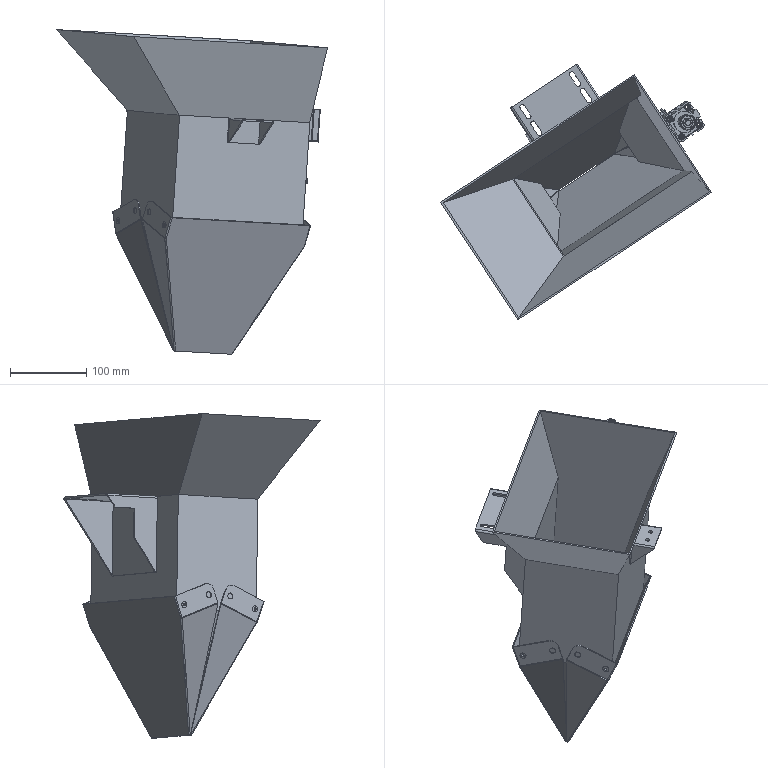Assembly | SolidWorks | mm | 21 component files | 21 solids | 784 faces | box 355.68 x 336.06 x 426.21 mm | volume 669723 mm3 | plane 339 | cylinder 308 | cone 109 | spline 16 | torus 10 | sphere 2 | commonest cylinder face diameters 8 x60 0.4 x46 7.9 x18 8.2 x16 4.917 x16 0.2 x12 6.5 x12 3.2 x9
Bill of materials:
BucketCylinderConnection | 1 | AISI 304 | Thin-wall formed bracket: a rectangular plate with four elongated slots, and side walls bent down along two opposite edges. The side walls have tapered, non-rectangular outlines.
DoorConnectionPiece | 2 | AISI 304 | Flat elongated link or strap with fully rounded ends and one round through-hole near each end.
DoorCylinderMount | 1 | AISI 304 | Thin L-shaped angle bracket. One leg is plain and rectangular. The other leg has a large central hole with four smaller holes arranged around it.
DoorFisheyeShaftPin | 1 |  | Headed bolt-like pin: a short head with flat faces on its sides, a plain cylindrical shank, and a section of external thread-like grooves at the free end.
DoorGasket | 4 |  | Plain cylindrical sleeve or spacer with a concentric round through-bore and flat ends.
F-M8X125U | 1 |  | Rod-end-style eye component: a rounded eye housing holding a separate-looking ring with a bore, a cylindrical shank, and a hexagonal collar with an axial bore at the end of the shank.
KnucklePin | 2 |  | Flanged bushing: a cylindrical body with a concentric through-bore, and a larger flange at one end that has at least one straight flat on its edge.
LinearGuideRodSheetMetal | 1 | AISI 304 | Thin formed channel-type bracket: a rectangular base plate with two round holes, and triangular walls bent up along two opposite edges.
MaterialChannel | 1 | AISI 304 | Thin open sheet-metal shape like a hopper or chute: an outward-flared rectangular upper rim, vertical walls below it, and tapered tabs or legs hanging from the lower edge.
MaterialGate | 2 | AISI 304 | Tapered open trough: a trapezoidal bottom panel with two inclined side walls narrowing toward one end. At the wide end there are bent-out end tabs, each with two round holes.
SDAJ-25x20_20b | 1 |  | Compact, roughly square prismatic block with chamfered corners and lengthwise extruded-profile grooves on its sides. Each end face has four corner through-holes with counterbores, a shallow circular recess or ring, and a raised central cylindrical boss with a central bore. The boss sticks out a little from both end faces. One side face has two small round ports.
Mates:
1. coincident | MaterialGate-1 face at (-298.666, 15.944, 688.726) dir (-0.8341, -0.5496, 0.04788) | MaterialGate-2 face at (-295.771, 11.528, 688.461) dir (-0.8341, -0.5496, 0.04788)
2. coincident | DoorConnectionPiece-1 face at (-101.704, 138.808, 740.065) dir (-0.8341, -0.5496, 0.04788) | DoorConnectionPiece-2 face at (-101.704, 138.808, 740.065) dir (0.8341, 0.5496, -0.04788)
3. concentric | KnucklePin-2 face at (-94.22, 126.738, 686.887) dir (-0.8341, -0.5496, 0.04788) r 4 | DoorConnectionPiece-1 face at (-96.017, 125.554, 686.99) dir (0.8341, 0.5496, -0.04788) r 4
4. concentric | KnucklePin-1 face at (-112.662, 154.873, 688.573) dir (-0.8341, -0.5496, 0.04788) r 4 | DoorConnectionPiece-2 face at (-116.128, 152.59, 688.772) dir (0.8341, 0.5496, -0.04788) r 4
5. coincident | MaterialChannel-1 face at (-315.723, 67.887, 831.179) dir (-0.5475, 0.8353, 0.05005) | BucketCylinderConnection-1 face at (-274.02, 95.366, 828.785) dir (0.5475, -0.8353, -0.05005)
6. coincident | MaterialChannel-1 face at (-144.74, 180.552, 821.364) dir (0.8341, 0.5496, -0.04788) | DoorCylinderMount-1 face at (-123.09, 145.425, 795.294) dir (-0.8341, -0.5496, 0.04788)
7. distance | BucketCylinderConnection-1 face at (-229.15, 218.226, 827.661) dir (0.8341, 0.5496, -0.04788) | MaterialChannel-1 face at (-144.74, 180.552, 821.364) dir (0.8341, 0.5496, -0.04788)
8. distance | DoorCylinderMount-1 face at (-99.938, 112.837, 793.221) dir (0.5475, -0.8353, -0.05005) | MaterialChannel-1 face at (-247.283, -36.525, 824.923) dir (0.5475, -0.8353, -0.05005)
9. coincident | MaterialChannel-1 face at (-315.723, 67.887, 831.179) dir (0.0675, -0.01553, 0.9976) | BucketCylinderConnection-1 face at (-229.15, 218.226, 827.661) dir (0.0675, -0.01553, 0.9976)
10. concentric | MaterialChannel-1 face at (-89.92, 84.239, 670.806) dir (-0.8341, -0.5496, 0.04788) r 4 | MaterialGate-2 face at (-84.915, 87.537, 670.519) dir (0.8341, 0.5496, -0.04788) r 4
11. concentric | MaterialChannel-1 face at (-150.695, 176.957, 676.362) dir (-0.8341, -0.5496, 0.04788) r 4 | MaterialGate-1 face at (-145.69, 180.254, 676.074) dir (0.8341, 0.5496, -0.04788) r 4
12. coincident | MaterialChannel-1 face at (-247.283, -36.525, 824.923) dir (0.5475, -0.8353, -0.05005) | LinearGuideRodSheetMetal-1 face at (-182.778, 6.099, 819.217) dir (-0.5475, 0.8353, 0.05005)
13. coincident | BucketCylinderConnection-1 face at (-229.15, 218.226, 827.661) dir (0.0675, -0.01553, 0.9976) | LinearGuideRodSheetMetal-1 face at (-181.548, 4.398, 821.112) dir (0.0675, -0.01553, 0.9976)
14. distance | MaterialChannel-1 face at (-144.74, 180.552, 821.364) dir (0.8341, 0.5496, -0.04788) | MaterialGate-1 face at (-116.423, 136.028, 678.264) dir (-0.8341, -0.5496, 0.04788)
15. distance | LinearGuideRodSheetMetal-1 face at (-181.683, 4.429, 819.117) dir (-0.8341, -0.5496, 0.04788) | MaterialChannel-1 face at (-315.723, 67.887, 831.179) dir (-0.8341, -0.5496, 0.04788)
16. concentric | MaterialChannel-1 face at (-89.92, 84.239, 670.806) dir (-0.8341, -0.5496, 0.04788) r 4 | DoorGasket-1 face at (-259.235, -27.327, 680.526) dir (-0.8341, -0.5496, 0.04788) r 4
17. concentric | MaterialChannel-1 face at (-150.695, 176.957, 676.362) dir (-0.8341, -0.5496, 0.04788) r 4 | DoorGasket-2 face at (-320.01, 65.391, 686.081) dir (-0.8341, -0.5496, 0.04788) r 4
18. coincident | MaterialChannel-1 face at (-312.96, 67.316, 830.983) dir (0.8341, 0.5496, -0.04788) | DoorGasket-2 face at (-320.01, 65.391, 686.081) dir (0.8341, 0.5496, -0.04788)
19. coincident | MaterialChannel-1 face at (-312.96, 67.316, 830.983) dir (0.8341, 0.5496, -0.04788) | DoorGasket-1 face at (-259.235, -27.327, 680.526) dir (0.8341, 0.5496, -0.04788)
20. concentric | MaterialChannel-1 face at (-89.92, 84.239, 670.806) dir (-0.8341, -0.5496, 0.04788) r 4 | DoorGasket-4 face at (-83.247, 88.636, 670.423) dir (-0.8341, -0.5496, 0.04788) r 4
21. concentric | MaterialChannel-1 face at (-150.695, 176.957, 676.362) dir (-0.8341, -0.5496, 0.04788) r 4 | DoorGasket-3 face at (-144.022, 181.353, 675.979) dir (-0.8341, -0.5496, 0.04788) r 4
22. coincident | MaterialChannel-1 face at (-145.313, 177.782, 821.359) dir (-0.8341, -0.5496, 0.04788) | DoorGasket-3 face at (-152.363, 175.857, 676.457) dir (-0.8341, -0.5496, 0.04788)
23. coincident | MaterialChannel-1 face at (-145.313, 177.782, 821.359) dir (-0.8341, -0.5496, 0.04788) | DoorGasket-4 face at (-91.588, 83.14, 670.902) dir (-0.8341, -0.5496, 0.04788)
24. concentric | DoorConnectionPiece-1 face at (-96.017, 125.554, 686.99) dir (0.8341, 0.5496, -0.04788) r 4 | KnucklePin-2 face at (-94.22, 126.738, 686.887) dir (-0.8341, -0.5496, 0.04788) r 4
25. coincident | MaterialGate-2 face at (-113.528, 131.612, 677.999) dir (-0.8341, -0.5496, 0.04788) | KnucklePin-2 face at (-105.063, 119.594, 687.509) dir (0.8341, 0.5496, -0.04788)
26. concentric | DoorConnectionPiece-2 face at (-116.128, 152.59, 688.772) dir (0.8341, 0.5496, -0.04788) r 4 | KnucklePin-1 face at (-112.662, 154.873, 688.573) dir (-0.8341, -0.5496, 0.04788) r 4
27. coincident | MaterialGate-1 face at (-116.423, 136.028, 678.264) dir (-0.8341, -0.5496, 0.04788) | KnucklePin-1 face at (-123.505, 147.729, 689.195) dir (0.8341, 0.5496, -0.04788)
28. coincident | DoorConnectionPiece-2 face at (-103.372, 137.709, 740.161) dir (-0.8341, -0.5496, 0.04788) | DoorFisheyeShaftPin-1 face at (-103.372, 137.709, 740.161) dir (0.8341, 0.5496, -0.04788)
29. distance | DoorCylinderMount-1 face at (-119.544, 145.721, 829.141) dir (0.0675, -0.01553, 0.9976) | BucketCylinderConnection-1 face at (-229.15, 218.226, 827.661) dir (0.0675, -0.01553, 0.9976)
30. concentric | DoorConnectionPiece-1 face at (-101.704, 138.808, 740.065) dir (0.8341, 0.5496, -0.04788) r 4 | DoorFisheyeShaftPin-1 face at (-89.193, 147.052, 739.347) dir (-0.8341, -0.5496, 0.04788) r 4
31. concentric | DoorConnectionPiece-2 face at (-103.372, 137.709, 740.161) dir (0.8341, 0.5496, -0.04788) r 4 | DoorFisheyeShaftPin-1 face at (-89.193, 147.052, 739.347) dir (-0.8341, -0.5496, 0.04788) r 4
32. concentric | MaterialGate-2 face at (-105.063, 119.594, 687.509) dir (0.8341, 0.5496, -0.04788) r 4 | KnucklePin-2 face at (-94.22, 126.738, 686.887) dir (-0.8341, -0.5496, 0.04788) r 4
33. concentric | MaterialGate-1 face at (-123.505, 147.729, 689.195) dir (0.8341, 0.5496, -0.04788) r 4 | KnucklePin-1 face at (-112.662, 154.873, 688.573) dir (-0.8341, -0.5496, 0.04788) r 4
34. concentric | DoorCylinderMount-1 face at (-91.288, 142.459, 793.096) dir (0.0675, -0.01553, 0.9976) r 9 | SDAJ25x20-20B(00)+()-1/SDAJ-25x20_20b-1 face at (-91.099, 142.415, 795.89) dir (-0.0675, 0.01553, -0.9976) r 8.5
35. concentric | DoorCylinderMount-1 face at (-71.946, 138.459, 791.725) dir (0.0675, -0.01553, 0.9976) r 3.15 | SDAJ25x20-20B(00)+()-1/SDAJ-25x20_20b-1 face at (-70.562, 138.14, 812.176) dir (-0.0675, 0.01553, -0.9976) r 4.1
36. coincident | DoorCylinderMount-1 face at (-85.557, 170.156, 793.14) dir (0.0675, -0.01553, 0.9976) | SDAJ25x20-20B(00)+()-1/SDAJ-25x20_20b-1 face at (-95.123, 163.614, 793.685) dir (-0.0675, 0.01553, -0.9976)
37. concentric | F-M8X125U-1 face at (-92.473, 142.731, 775.589) dir (-0.0675, 0.01553, -0.9976) r 3.324 | SDAJ25x20-20B(00)+()-1/SDAJ-25x20-B2020_r-1 face at (-89.229, 141.985, 823.523) dir (-0.0675, 0.01553, -0.9976) r 4
38. distance | F-M8X125U-1 face at (-98.728, 138.609, 775.948) dir (0.0675, -0.01553, 0.9976) | SDAJ25x20-20B(00)+()-1/SDAJ-25- M8x1_25-1 face at (-92.068, 142.638, 781.574) dir (0.0675, -0.01553, 0.9976)
39. concentric | DoorFisheyeShaftPin-1 face at (-89.193, 147.052, 739.347) dir (-0.8341, -0.5496, 0.04788) r 4 | F-M8X125U-1 face at (-89.898, 146.588, 739.388) dir (-0.8341, -0.5496, 0.04788) r 4
40. coincident | SDAJ-25x20_20b-1 axis at (-80.9, 0, 0) dir (1, 0, 0) | SDAJ-25x20-B2020_r-1 axis at (80.9, 0, 0) dir (-1, 0, 0)
41. angle | SDAJ-25x20-B2020_r-1 plane at (0, 0, 0) dir (0, 0, -1) | SDAJ-25x20_20b-1 plane at (0, 0, 0) dir (0, 1, 0)
42. coincident | SDAJ-25x20-B2020_r-1 axis at (-80.9, 0, 0) dir (1, 0, 0) | SDAJ-25- M8x1_25-1 axis at (-92.45, 0, 0) dir (1, 0, 0)
43. angle | SDAJ-25- M8x1_25-1 plane at (-11.55, 0, 0) dir (0, 0, -1) | SDAJ-25x20-B2020_r-1 plane at (0, 0, 0) dir (0, 0, -1)
44. distance | SDA-25-M8x1_2520 - A_Nut-1 plane at (102, 0, 0) dir (-1, 0, 0) | SDAJ-25x20-B2020_r-1 plane at (102, 0, 0) dir (1, 0, 0)
45. coincident | SDAJ-25x20-B2020_r-1 axis at (80.9, 0, 0) dir (-1, 0, 0) | SDA-25-M8x1_2520 - A_Nut-1 axis at (21.1, 0, 0) dir (1, 0, 0)
46. angle | SDA-25-M8x1_2520 - A_Nut-1 plane at (102, 0, 0) dir (0, 0, -1) | SDAJ-25x20-B2020_r-1 plane at (0, 0, 0) dir (0, 0, -1)
47. distance | SDAJ-25- M8x1_25SDAJ_NUT-1 plane at (105, 0, 0) dir (-1, 0, 0) | SDAJ-25x20-B2020_r-1 plane at (102, 0, 0) dir (1, 0, 0)
48. coincident | SDAJ-25x20-B2020_r-1 axis at (80.9, 0, 0) dir (-1, 0, 0) | SDAJ-25- M8x1_25SDAJ_NUT-1 axis at (27.1, 0, 0) dir (1, 0, 0)
49. angle | SDAJ-25- M8x1_25SDAJ_NUT-1 plane at (108, 0, 0) dir (0, 0, -1) | SDAJ-25x20-B2020_r-1 plane at (0, 0, 0) dir (0, 0, -1)